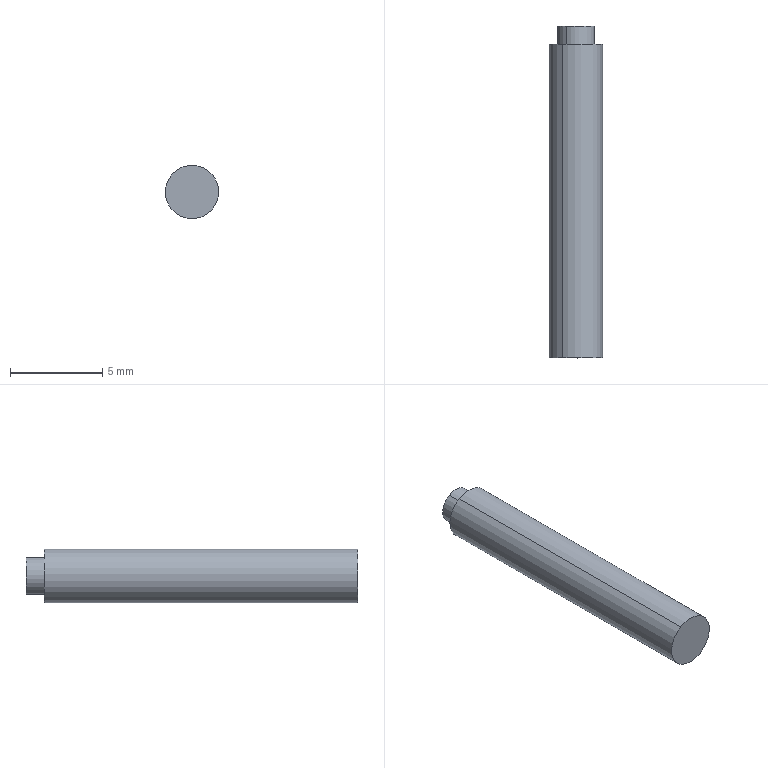Component | SolidWorks | DCRSW-310-ReflectionFiber-1 | 1 solid | 7 faces | box 2.9 x 18 x 2.9 mm | volume 115 mm3 | cylinder 4 | plane 3 | commonest cylinder face diameters 2.9 x2 2 x2
build123d program:
from build123d import *

# Parameters (mm, degrees)
SKETCH1_R           = 1
BOSS_EXTRUDE1_DEPTH = 1
SKETCH2_R           = 1.45
BOSS_EXTRUDE2_DEPTH = 17


with BuildPart() as part:
    # Sketch1 → Boss-Extrude1 (new body)
    with BuildSketch(Plane(origin=(0, 0, 0), x_dir=(1, 0, 0), z_dir=(0, 1, 0))):
        with Locations(Location((0, 0, 0), (0, 0, 270))):
            Circle(SKETCH1_R)
    extrude(amount=BOSS_EXTRUDE1_DEPTH)

    # Sketch2 → Boss-Extrude2 (add)
    with BuildSketch(Plane(origin=(0, 1, 0), x_dir=(1, 0, 0), z_dir=(0, 1, 0))):
        with Locations(Location((0, 0, 0), (0, 0, 270))):
            Circle(SKETCH2_R)
    extrude(amount=BOSS_EXTRUDE2_DEPTH)


solid = part.part

# Placed as in the assembly
solid = solid.moved(Location((13, 14, 172.5), (180, 0, 0)))
STEP:
#1=COLOUR_RGB('',0.7922,0.8196,0.9333);
#2=FILL_AREA_STYLE_COLOUR('',#1);
#3=FILL_AREA_STYLE('',(#2));
#4=SURFACE_STYLE_FILL_AREA(#3);
#5=SURFACE_SIDE_STYLE('',(#4));
#6=SURFACE_STYLE_USAGE(.BOTH.,#5);
#7=PRESENTATION_STYLE_ASSIGNMENT((#6));
#8=CARTESIAN_POINT('',(0.541,-0.1575,6.742));
#9=VERTEX_POINT('',#8);
#10=CARTESIAN_POINT('',(0.4826,-0.1575,6.84));
#11=VERTEX_POINT('',#10);
#12=CARTESIAN_POINT('',(0.5118,-0.1575,6.791));
#13=DIRECTION('',(-0.,-1.,0.));
#14=DIRECTION('',(0.512,0.,-0.859));
#15=AXIS2_PLACEMENT_3D('',#12,#13,#14);
#16=CIRCLE('',#15,0.05709);
#17=EDGE_CURVE('',#9,#11,#16,.T.);
#18=ORIENTED_EDGE('',*,*,#17,.F.);
#19=CARTESIAN_POINT('',(0.541,0.5118,6.742));
#20=VERTEX_POINT('',#19);
#21=CARTESIAN_POINT('',(0.541,-0.1575,6.742));
#22=DIRECTION('',(0.,1.,-0.));
#23=VECTOR('',#22,39.37);
#24=LINE('',#21,#23);
#25=EDGE_CURVE('',#9,#20,#24,.T.);
#26=ORIENTED_EDGE('',*,*,#25,.T.);
#27=CARTESIAN_POINT('',(0.4826,0.5118,6.84));
#28=VERTEX_POINT('',#27);
#29=CARTESIAN_POINT('',(0.5118,0.5118,6.791));
#30=DIRECTION('',(-0.,-1.,0.));
#31=DIRECTION('',(0.512,0.,-0.859));
#32=AXIS2_PLACEMENT_3D('',#29,#30,#31);
#33=CIRCLE('',#32,0.05709);
#34=EDGE_CURVE('',#20,#28,#33,.T.);
#35=ORIENTED_EDGE('',*,*,#34,.T.);
#36=CARTESIAN_POINT('',(0.4826,-0.1575,6.84));
#37=DIRECTION('',(0.,1.,-0.));
#38=VECTOR('',#37,39.37);
#39=LINE('',#36,#38);
#40=EDGE_CURVE('',#11,#28,#39,.T.);
#41=ORIENTED_EDGE('',*,*,#40,.F.);
#42=EDGE_LOOP('',(#18,#26,#35,#41));
#43=FACE_OUTER_BOUND('',#42,.T.);
#44=CARTESIAN_POINT('',(0.5118,-0.1575,6.791));
#45=DIRECTION('',(0.,1.,-0.));
#46=DIRECTION('',(-0.512,0.,0.859));
#47=AXIS2_PLACEMENT_3D('',#44,#45,#46);
#48=CYLINDRICAL_SURFACE('',#47,0.05709);
#49=ADVANCED_FACE('',(#43),#48,.T.);
#50=CARTESIAN_POINT('',(0.532,0.5118,6.758));
#51=VERTEX_POINT('',#50);
#52=CARTESIAN_POINT('',(0.4917,0.5118,6.825));
#53=VERTEX_POINT('',#52);
#54=CARTESIAN_POINT('',(0.5118,0.5118,6.791));
#55=DIRECTION('',(-0.,-1.,0.));
#56=DIRECTION('',(0.512,0.,-0.859));
#57=AXIS2_PLACEMENT_3D('',#54,#55,#56);
#58=CIRCLE('',#57,0.03937);
#59=EDGE_CURVE('',#51,#53,#58,.T.);
#60=ORIENTED_EDGE('',*,*,#59,.F.);
#61=CARTESIAN_POINT('',(0.532,0.5512,6.758));
#62=VERTEX_POINT('',#61);
#63=CARTESIAN_POINT('',(0.532,0.5118,6.758));
#64=DIRECTION('',(0.,1.,-0.));
#65=VECTOR('',#64,39.37);
#66=LINE('',#63,#65);
#67=EDGE_CURVE('',#51,#62,#66,.T.);
#68=ORIENTED_EDGE('',*,*,#67,.T.);
#69=CARTESIAN_POINT('',(0.4917,0.5512,6.825));
#70=VERTEX_POINT('',#69);
#71=CARTESIAN_POINT('',(0.5118,0.5512,6.791));
#72=DIRECTION('',(-0.,-1.,0.));
#73=DIRECTION('',(0.512,0.,-0.859));
#74=AXIS2_PLACEMENT_3D('',#71,#72,#73);
#75=CIRCLE('',#74,0.03937);
#76=EDGE_CURVE('',#62,#70,#75,.T.);
#77=ORIENTED_EDGE('',*,*,#76,.T.);
#78=CARTESIAN_POINT('',(0.4917,0.5118,6.825));
#79=DIRECTION('',(0.,1.,-0.));
#80=VECTOR('',#79,39.37);
#81=LINE('',#78,#80);
#82=EDGE_CURVE('',#53,#70,#81,.T.);
#83=ORIENTED_EDGE('',*,*,#82,.F.);
#84=EDGE_LOOP('',(#60,#68,#77,#83));
#85=FACE_OUTER_BOUND('',#84,.T.);
#86=CARTESIAN_POINT('',(0.5118,0.5118,6.791));
#87=DIRECTION('',(0.,1.,-0.));
#88=DIRECTION('',(-0.512,0.,0.859));
#89=AXIS2_PLACEMENT_3D('',#86,#87,#88);
#90=CYLINDRICAL_SURFACE('',#89,0.03937);
#91=ADVANCED_FACE('',(#85),#90,.T.);
#92=ORIENTED_EDGE('',*,*,#67,.F.);
#93=CARTESIAN_POINT('',(0.5118,0.5118,6.791));
#94=DIRECTION('',(-0.,-1.,0.));
#95=DIRECTION('',(0.512,0.,-0.859));
#96=AXIS2_PLACEMENT_3D('',#93,#94,#95);
#97=CIRCLE('',#96,0.03937);
#98=EDGE_CURVE('',#53,#51,#97,.T.);
#99=ORIENTED_EDGE('',*,*,#98,.F.);
#100=ORIENTED_EDGE('',*,*,#82,.T.);
#101=CARTESIAN_POINT('',(0.5118,0.5512,6.791));
#102=DIRECTION('',(-0.,-1.,0.));
#103=DIRECTION('',(0.512,0.,-0.859));
#104=AXIS2_PLACEMENT_3D('',#101,#102,#103);
#105=CIRCLE('',#104,0.03937);
#106=EDGE_CURVE('',#70,#62,#105,.T.);
#107=ORIENTED_EDGE('',*,*,#106,.T.);
#108=EDGE_LOOP('',(#92,#99,#100,#107));
#109=FACE_OUTER_BOUND('',#108,.T.);
#110=CARTESIAN_POINT('',(0.5118,0.5118,6.791));
#111=DIRECTION('',(0.,1.,-0.));
#112=DIRECTION('',(-0.512,0.,0.859));
#113=AXIS2_PLACEMENT_3D('',#110,#111,#112);
#114=CYLINDRICAL_SURFACE('',#113,0.03937);
#115=ADVANCED_FACE('',(#109),#114,.T.);
#116=ORIENTED_EDGE('',*,*,#106,.F.);
#117=ORIENTED_EDGE('',*,*,#76,.F.);
#118=EDGE_LOOP('',(#116,#117));
#119=FACE_OUTER_BOUND('',#118,.T.);
#120=CARTESIAN_POINT('',(0.5118,0.5512,6.791));
#121=DIRECTION('',(0.,-1.,0.));
#122=DIRECTION('',(0.512,-0.,-0.859));
#123=AXIS2_PLACEMENT_3D('',#120,#121,#122);
#124=PLANE('',#123);
#125=ADVANCED_FACE('',(#119),#124,.F.);
#126=ORIENTED_EDGE('',*,*,#25,.F.);
#127=CARTESIAN_POINT('',(0.5118,-0.1575,6.791));
#128=DIRECTION('',(-0.,-1.,0.));
#129=DIRECTION('',(0.512,0.,-0.859));
#130=AXIS2_PLACEMENT_3D('',#127,#128,#129);
#131=CIRCLE('',#130,0.05709);
#132=EDGE_CURVE('',#11,#9,#131,.T.);
#133=ORIENTED_EDGE('',*,*,#132,.F.);
#134=ORIENTED_EDGE('',*,*,#40,.T.);
#135=CARTESIAN_POINT('',(0.5118,0.5118,6.791));
#136=DIRECTION('',(-0.,-1.,0.));
#137=DIRECTION('',(0.512,0.,-0.859));
#138=AXIS2_PLACEMENT_3D('',#135,#136,#137);
#139=CIRCLE('',#138,0.05709);
#140=EDGE_CURVE('',#28,#20,#139,.T.);
#141=ORIENTED_EDGE('',*,*,#140,.T.);
#142=EDGE_LOOP('',(#126,#133,#134,#141));
#143=FACE_OUTER_BOUND('',#142,.T.);
#144=CARTESIAN_POINT('',(0.5118,-0.1575,6.791));
#145=DIRECTION('',(0.,1.,-0.));
#146=DIRECTION('',(-0.512,0.,0.859));
#147=AXIS2_PLACEMENT_3D('',#144,#145,#146);
#148=CYLINDRICAL_SURFACE('',#147,0.05709);
#149=ADVANCED_FACE('',(#143),#148,.T.);
#150=ORIENTED_EDGE('',*,*,#132,.T.);
#151=ORIENTED_EDGE('',*,*,#17,.T.);
#152=EDGE_LOOP('',(#150,#151));
#153=FACE_OUTER_BOUND('',#152,.T.);
#154=CARTESIAN_POINT('',(0.5118,-0.1575,6.791));
#155=DIRECTION('',(0.,-1.,0.));
#156=DIRECTION('',(0.512,-0.,-0.859));
#157=AXIS2_PLACEMENT_3D('',#154,#155,#156);
#158=PLANE('',#157);
#159=ADVANCED_FACE('',(#153),#158,.T.);
#160=ORIENTED_EDGE('',*,*,#98,.T.);
#161=ORIENTED_EDGE('',*,*,#59,.T.);
#162=EDGE_LOOP('',(#160,#161));
#163=FACE_BOUND('',#162,.T.);
#164=ORIENTED_EDGE('',*,*,#140,.F.);
#165=ORIENTED_EDGE('',*,*,#34,.F.);
#166=EDGE_LOOP('',(#164,#165));
#167=FACE_OUTER_BOUND('',#166,.T.);
#168=CARTESIAN_POINT('',(0.5118,0.5118,6.791));
#169=DIRECTION('',(0.,-1.,0.));
#170=DIRECTION('',(0.512,-0.,-0.859));
#171=AXIS2_PLACEMENT_3D('',#168,#169,#170);
#172=PLANE('',#171);
#173=ADVANCED_FACE('',(#163,#167),#172,.F.);
#174=CLOSED_SHELL('',(#49,#91,#115,#125,#149,#159,#173));
#175=MANIFOLD_SOLID_BREP('',#174);
#176=STYLED_ITEM('',(#7),#175);
#177=(LENGTH_UNIT()NAMED_UNIT(*)SI_UNIT($,.METRE.));
#178=LENGTH_MEASURE_WITH_UNIT(LENGTH_MEASURE(0.0254),#177);
#179=DIMENSIONAL_EXPONENTS(1.,0.,0.,0.,0.,0.,0.);
#180=(CONVERSION_BASED_UNIT('',#178)LENGTH_UNIT()NAMED_UNIT(#179));
#181=UNCERTAINTY_MEASURE_WITH_UNIT(LENGTH_MEASURE(0.00001),#180,'','');
#182=(NAMED_UNIT(*)PLANE_ANGLE_UNIT()SI_UNIT($,.RADIAN.));
#183=(NAMED_UNIT(*)SI_UNIT($,.STERADIAN.)SOLID_ANGLE_UNIT());
#184=(GEOMETRIC_REPRESENTATION_CONTEXT(3)GLOBAL_UNCERTAINTY_ASSIGNED_CONTEXT((#181))GLOBAL_UNIT_ASSIGNED_CONTEXT((#180,#182,#183))REPRESENTATION_CONTEXT('',''));
#185=MECHANICAL_DESIGN_GEOMETRIC_PRESENTATION_REPRESENTATION('',(#176),#184);
#186=PRESENTATION_LAYER_ASSIGNMENT('','',(#176));
#187=CARTESIAN_POINT('',(0.,0.,0.));
#188=DIRECTION('',(0.,0.,1.));
#189=DIRECTION('',(1.,0.,0.));
#190=AXIS2_PLACEMENT_3D('',#187,#188,#189);
#191=(LENGTH_UNIT()NAMED_UNIT(*)SI_UNIT($,.METRE.));
#192=LENGTH_MEASURE_WITH_UNIT(LENGTH_MEASURE(0.0254),#191);
#193=DIMENSIONAL_EXPONENTS(1.,0.,0.,0.,0.,0.,0.);
#194=(CONVERSION_BASED_UNIT('',#192)LENGTH_UNIT()NAMED_UNIT(#193));
#195=UNCERTAINTY_MEASURE_WITH_UNIT(LENGTH_MEASURE(0.00001),#194,'','');
#196=(NAMED_UNIT(*)PLANE_ANGLE_UNIT()SI_UNIT($,.RADIAN.));
#197=(NAMED_UNIT(*)SI_UNIT($,.STERADIAN.)SOLID_ANGLE_UNIT());
#198=(GEOMETRIC_REPRESENTATION_CONTEXT(3)GLOBAL_UNCERTAINTY_ASSIGNED_CONTEXT((#195))GLOBAL_UNIT_ASSIGNED_CONTEXT((#194,#196,#197))REPRESENTATION_CONTEXT('',''));
#199=ADVANCED_BREP_SHAPE_REPRESENTATION('',(#175,#190),#198);